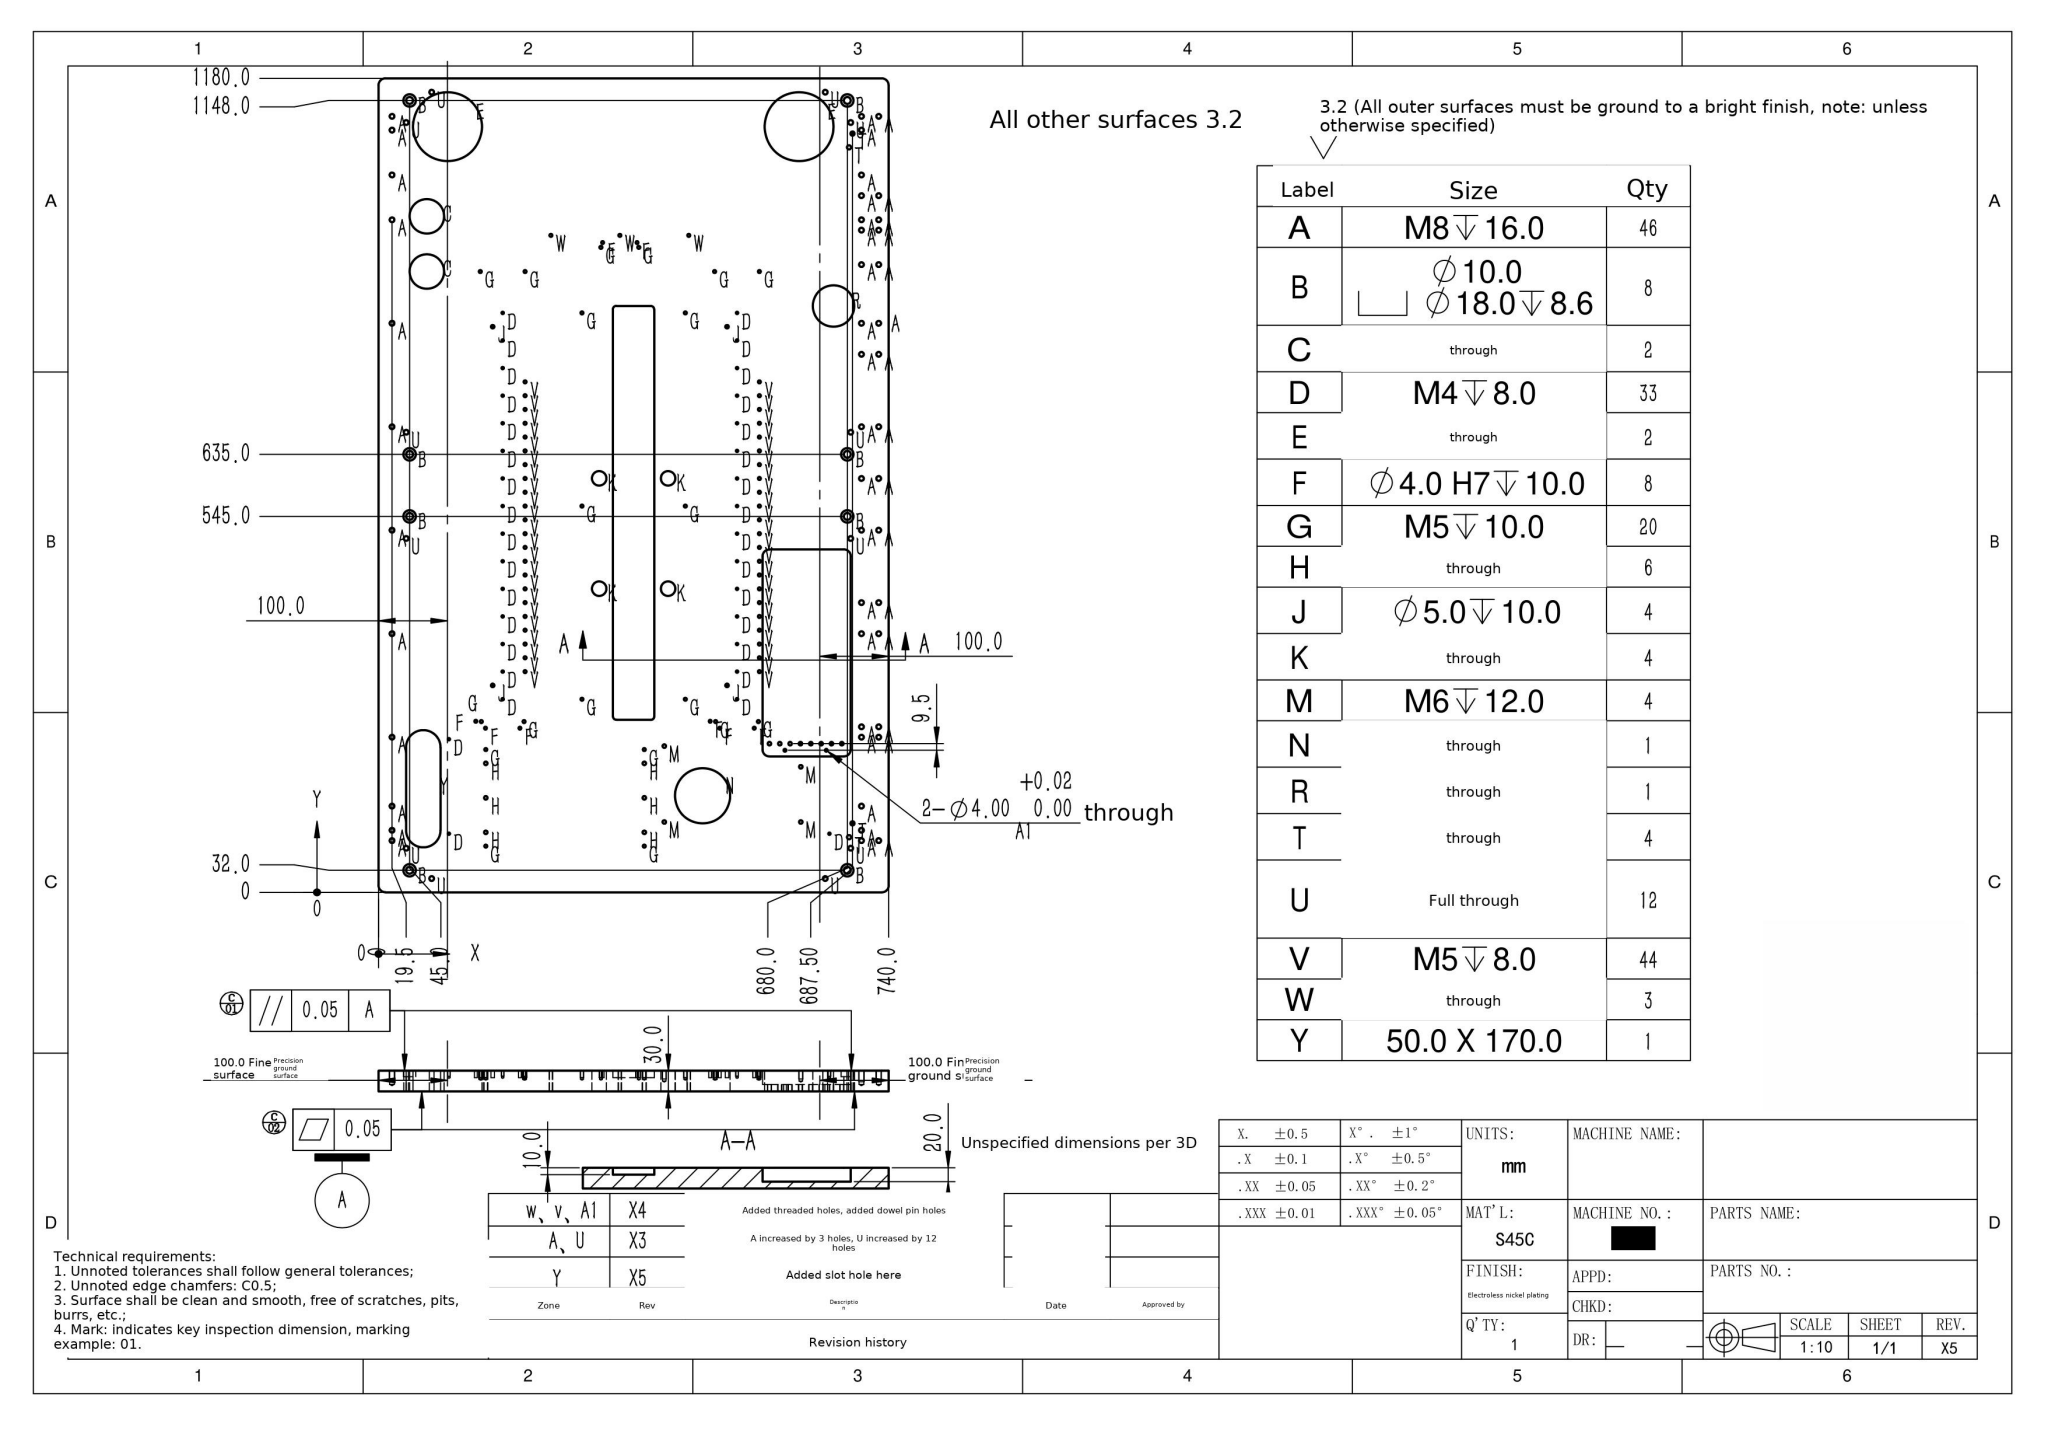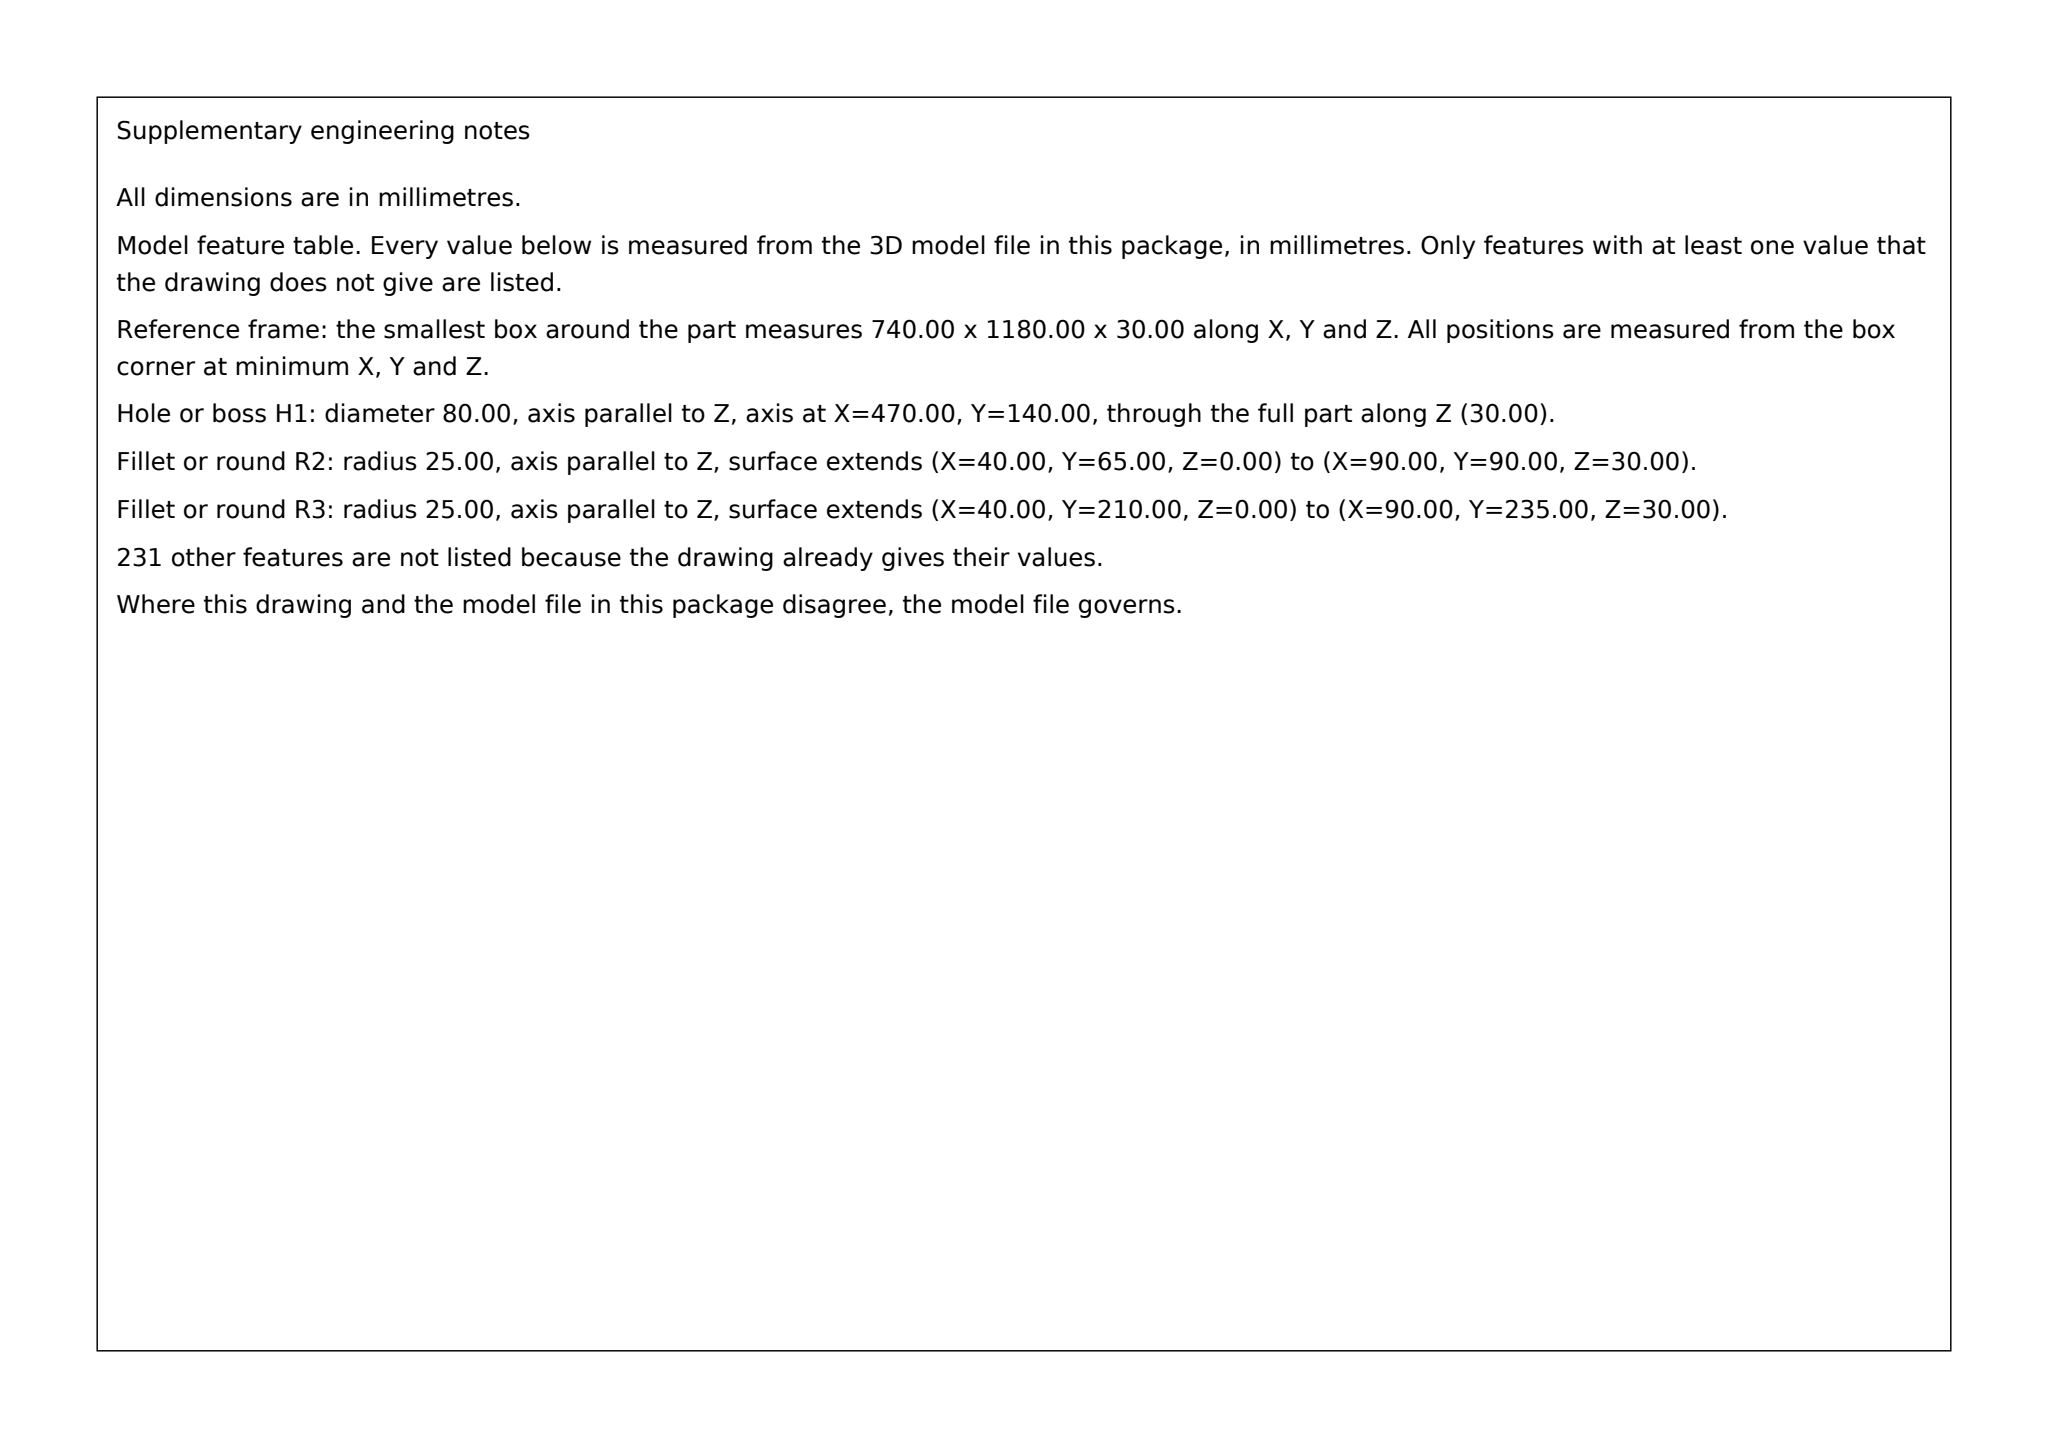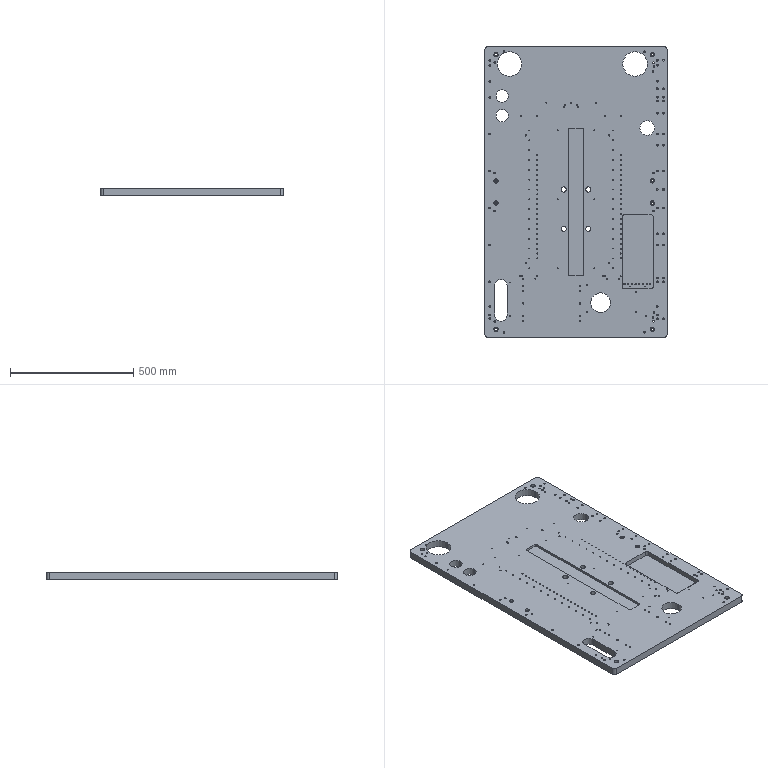Part | SolidWorks | mm | material S45C | 1 solid | 786 faces | box 740 x 1180 x 30 mm | volume 23857964 mm3 | cylinder 454 | cone 294 | plane 38 | commonest cylinder face diameters 4.2 x134 6.8 x116 3.3 x66 5 x44 4 x20 10 x20 18 x16 21 x8